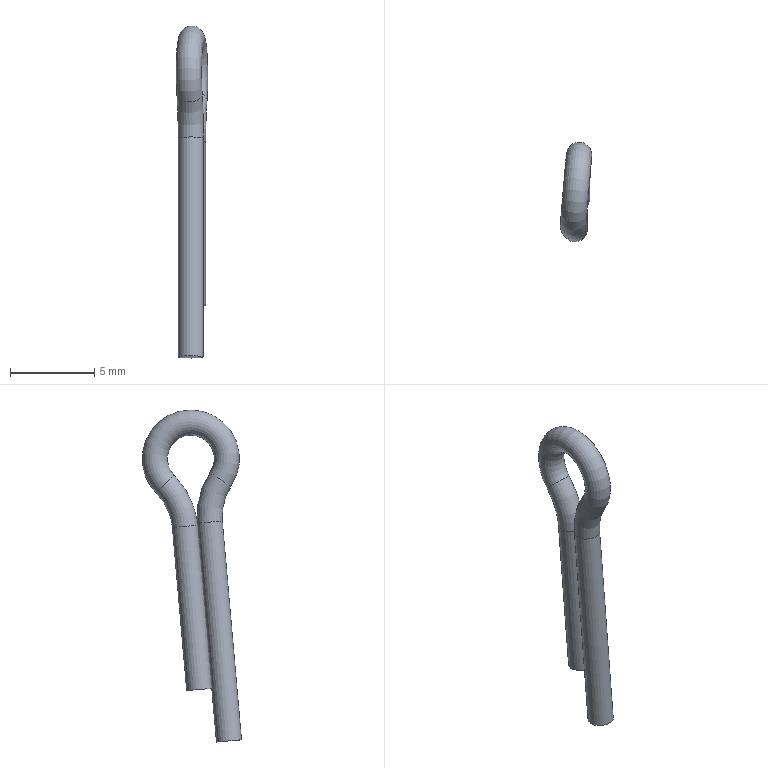Component | NX | COTTER_PIN | 1 solid | 7 faces | box 1.87 x 5.91 x 19.73 mm | volume 67 mm3 | torus 3 | cylinder 2 | plane 2 | commonest cylinder face diameters 1.5 x2
STEP:
#1=CARTESIAN_POINT('',(0.,0.,0.));
#2=DIRECTION('',(0.,0.,1.));
#3=DIRECTION('',(1.,0.,0.));
#4=AXIS2_PLACEMENT_3D('',#1,#2,#3);
#5=CARTESIAN_POINT('',(276.072,467.87,-17.811));
#6=VERTEX_POINT('',#5);
#7=CARTESIAN_POINT('',(276.006,467.126,-17.746));
#8=DIRECTION('',(0.,-0.08716,-0.9962));
#9=DIRECTION('',(0.08716,0.9924,-0.08682));
#10=AXIS2_PLACEMENT_3D('',#7,#8,#9);
#11=CIRCLE('',#10,0.75);
#12=CARTESIAN_POINT('',(276.006,467.126,-17.746));
#13=DIRECTION('',(0.,-0.08716,-0.9962));
#14=DIRECTION('',(0.08716,0.9924,-0.08682));
#15=AXIS2_PLACEMENT_3D('',#12,#13,#14);
#16=CYLINDRICAL_SURFACE('',#15,0.75);
#17=CARTESIAN_POINT('',(0.,-0.));
#18=DIRECTION('',(1.,0.));
#19=VECTOR('',#18,1.);
#20=LINE('',#17,#19);
#21=(GEOMETRIC_REPRESENTATION_CONTEXT(2)PARAMETRIC_REPRESENTATION_CONTEXT()REPRESENTATION_CONTEXT('',''));
#22=DEFINITIONAL_REPRESENTATION('',(#20),#21);
#23=PCURVE('',#16,#22);
#24=CARTESIAN_POINT('',(276.355,471.095,-18.094));
#25=DIRECTION('',(0.9962,-0.08682,0.007596));
#26=DIRECTION('',(0.,-0.08716,-0.9962));
#27=AXIS2_PLACEMENT_3D('',#24,#25,#26);
#28=TOROIDAL_SURFACE('',#27,4.,0.75);
#29=CARTESIAN_POINT('',(4.712,9.425));
#30=DIRECTION('',(0.,-1.));
#31=VECTOR('',#30,1.);
#32=LINE('',#29,#31);
#33=(GEOMETRIC_REPRESENTATION_CONTEXT(2)PARAMETRIC_REPRESENTATION_CONTEXT()REPRESENTATION_CONTEXT('',''));
#34=DEFINITIONAL_REPRESENTATION('',(#32),#33);
#35=PCURVE('',#28,#34);
#36=SURFACE_CURVE('',#11,(#23,#35),.PCURVE_S1.);
#37=EDGE_CURVE('',#6,#6,#36,.T.);
#38=ORIENTED_EDGE('',*,*,#37,.T.);
#39=CARTESIAN_POINT('',(276.072,467.022,-27.508));
#40=VERTEX_POINT('',#39);
#41=CARTESIAN_POINT('',(276.072,467.87,-17.811));
#42=CARTESIAN_POINT('',(276.072,467.022,-27.508));
#43=B_SPLINE_CURVE_WITH_KNOTS('',1,(#41,#42),.UNSPECIFIED.,.F.,.F.,(2,2),(-0.,9.734),.PIECEWISE_BEZIER_KNOTS.);
#44=CARTESIAN_POINT('',(6.283,0.));
#45=DIRECTION('',(0.,1.));
#46=VECTOR('',#45,1.);
#47=LINE('',#44,#46);
#48=(GEOMETRIC_REPRESENTATION_CONTEXT(2)PARAMETRIC_REPRESENTATION_CONTEXT()REPRESENTATION_CONTEXT('',''));
#49=DEFINITIONAL_REPRESENTATION('',(#47),#48);
#50=PCURVE('',#16,#49);
#51=CARTESIAN_POINT('',(0.,0.));
#52=DIRECTION('',(0.,1.));
#53=VECTOR('',#52,1.);
#54=LINE('',#51,#53);
#55=(GEOMETRIC_REPRESENTATION_CONTEXT(2)PARAMETRIC_REPRESENTATION_CONTEXT()REPRESENTATION_CONTEXT('',''));
#56=DEFINITIONAL_REPRESENTATION('',(#54),#55);
#57=PCURVE('',#16,#56);
#58=SEAM_CURVE('',#43,(#50,#57),.PCURVE_S1.);
#59=EDGE_CURVE('',#6,#40,#58,.T.);
#60=ORIENTED_EDGE('',*,*,#59,.T.);
#61=CARTESIAN_POINT('',(276.006,466.277,-27.443));
#62=DIRECTION('',(0.,-0.08716,-0.9962));
#63=DIRECTION('',(0.08716,0.9924,-0.08682));
#64=AXIS2_PLACEMENT_3D('',#61,#62,#63);
#65=CIRCLE('',#64,0.75);
#66=CARTESIAN_POINT('',(0.,9.734));
#67=DIRECTION('',(1.,0.));
#68=VECTOR('',#67,1.);
#69=LINE('',#66,#68);
#70=(GEOMETRIC_REPRESENTATION_CONTEXT(2)PARAMETRIC_REPRESENTATION_CONTEXT()REPRESENTATION_CONTEXT('',''));
#71=DEFINITIONAL_REPRESENTATION('',(#69),#70);
#72=PCURVE('',#16,#71);
#73=CARTESIAN_POINT('',(276.006,466.277,-27.443));
#74=DIRECTION('',(0.,-0.08716,-0.9962));
#75=DIRECTION('',(0.08716,0.9924,-0.08682));
#76=AXIS2_PLACEMENT_3D('',#73,#74,#75);
#77=PLANE('',#76);
#78=CARTESIAN_POINT('',(0.,0.));
#79=DIRECTION('',(1.,0.));
#80=AXIS2_PLACEMENT_2D('',#78,#79);
#81=CIRCLE('',#80,0.75);
#82=(GEOMETRIC_REPRESENTATION_CONTEXT(2)PARAMETRIC_REPRESENTATION_CONTEXT()REPRESENTATION_CONTEXT('',''));
#83=DEFINITIONAL_REPRESENTATION('',(#81),#82);
#84=PCURVE('',#77,#83);
#85=SURFACE_CURVE('',#65,(#72,#84),.PCURVE_S1.);
#86=EDGE_CURVE('',#40,#40,#85,.T.);
#87=ORIENTED_EDGE('',*,*,#86,.F.);
#88=ORIENTED_EDGE('',*,*,#59,.F.);
#89=EDGE_LOOP('',(#38,#60,#87,#88));
#90=FACE_BOUND('',#89,.T.);
#91=ADVANCED_FACE('',(#90),#16,.T.);
#92=CARTESIAN_POINT('',(276.139,468.813,-15.79));
#93=VERTEX_POINT('',#92);
#94=CARTESIAN_POINT('',(276.089,468.286,-15.258));
#95=DIRECTION('',(-0.05621,-0.7067,-0.7053));
#96=DIRECTION('',(0.06661,0.7022,-0.7088));
#97=AXIS2_PLACEMENT_3D('',#94,#95,#96);
#98=CIRCLE('',#97,0.75);
#99=CARTESIAN_POINT('',(4.011,9.425));
#100=DIRECTION('',(0.,-1.));
#101=VECTOR('',#100,1.);
#102=LINE('',#99,#101);
#103=(GEOMETRIC_REPRESENTATION_CONTEXT(2)PARAMETRIC_REPRESENTATION_CONTEXT()REPRESENTATION_CONTEXT('',''));
#104=DEFINITIONAL_REPRESENTATION('',(#102),#103);
#105=PCURVE('',#28,#104);
#106=CARTESIAN_POINT('',(275.945,466.777,-13.734));
#107=DIRECTION('',(-0.9962,0.08682,-0.007596));
#108=DIRECTION('',(-0.,0.08716,0.9962));
#109=AXIS2_PLACEMENT_3D('',#106,#107,#108);
#110=TOROIDAL_SURFACE('',#109,2.15,0.75);
#111=CARTESIAN_POINT('',(8.555,6.283));
#112=DIRECTION('',(0.,-1.));
#113=VECTOR('',#112,1.);
#114=LINE('',#111,#113);
#115=(GEOMETRIC_REPRESENTATION_CONTEXT(2)PARAMETRIC_REPRESENTATION_CONTEXT()REPRESENTATION_CONTEXT('',''));
#116=DEFINITIONAL_REPRESENTATION('',(#114),#115);
#117=PCURVE('',#110,#116);
#118=SURFACE_CURVE('',#98,(#105,#117),.PCURVE_S1.);
#119=EDGE_CURVE('',#93,#93,#118,.T.);
#120=ORIENTED_EDGE('',*,*,#119,.T.);
#121=CARTESIAN_POINT('',(276.139,468.813,-15.79));
#122=CARTESIAN_POINT('',(276.117,468.544,-16.059));
#123=CARTESIAN_POINT('',(276.099,468.313,-16.364));
#124=CARTESIAN_POINT('',(276.086,468.127,-16.7));
#125=CARTESIAN_POINT('',(276.077,467.989,-17.058));
#126=CARTESIAN_POINT('',(276.072,467.903,-17.432));
#127=CARTESIAN_POINT('',(276.072,467.87,-17.811));
#128=(BOUNDED_CURVE()B_SPLINE_CURVE(6,(#121,#122,#123,#124,#125,#126,#127),.UNSPECIFIED.,.F.,.F.)B_SPLINE_CURVE_WITH_KNOTS((7,7),(4.011,4.712),.PIECEWISE_BEZIER_KNOTS.)CURVE()GEOMETRIC_REPRESENTATION_ITEM()RATIONAL_B_SPLINE_CURVE((1.006,1.002,0.9996,0.9988,0.9996,1.002,1.006))REPRESENTATION_ITEM(''));
#129=CARTESIAN_POINT('',(0.,3.142));
#130=DIRECTION('',(1.,0.));
#131=VECTOR('',#130,1.);
#132=LINE('',#129,#131);
#133=(GEOMETRIC_REPRESENTATION_CONTEXT(2)PARAMETRIC_REPRESENTATION_CONTEXT()REPRESENTATION_CONTEXT('',''));
#134=DEFINITIONAL_REPRESENTATION('',(#132),#133);
#135=PCURVE('',#28,#134);
#136=CARTESIAN_POINT('',(0.,9.425));
#137=DIRECTION('',(1.,0.));
#138=VECTOR('',#137,1.);
#139=LINE('',#136,#138);
#140=(GEOMETRIC_REPRESENTATION_CONTEXT(2)PARAMETRIC_REPRESENTATION_CONTEXT()REPRESENTATION_CONTEXT('',''));
#141=DEFINITIONAL_REPRESENTATION('',(#139),#140);
#142=PCURVE('',#28,#141);
#143=SEAM_CURVE('',#128,(#135,#142),.PCURVE_S1.);
#144=EDGE_CURVE('',#93,#6,#143,.T.);
#145=ORIENTED_EDGE('',*,*,#144,.T.);
#146=ORIENTED_EDGE('',*,*,#37,.F.);
#147=ORIENTED_EDGE('',*,*,#144,.F.);
#148=EDGE_LOOP('',(#120,#145,#146,#147));
#149=FACE_BOUND('',#148,.T.);
#150=ADVANCED_FACE('',(#149),#28,.T.);
#151=CARTESIAN_POINT('',(275.748,464.372,-15.344));
#152=VERTEX_POINT('',#151);
#153=CARTESIAN_POINT('',(275.799,464.994,-14.927));
#154=DIRECTION('',(-0.05449,-0.5524,0.8318));
#155=DIRECTION('',(-0.06802,-0.829,-0.555));
#156=AXIS2_PLACEMENT_3D('',#153,#154,#155);
#157=CIRCLE('',#156,0.75);
#158=CARTESIAN_POINT('',(4.037,6.283));
#159=DIRECTION('',(0.,-1.));
#160=VECTOR('',#159,1.);
#161=LINE('',#158,#160);
#162=(GEOMETRIC_REPRESENTATION_CONTEXT(2)PARAMETRIC_REPRESENTATION_CONTEXT()REPRESENTATION_CONTEXT('',''));
#163=DEFINITIONAL_REPRESENTATION('',(#161),#162);
#164=PCURVE('',#110,#163);
#165=CARTESIAN_POINT('',(275.527,461.678,-17.148));
#166=DIRECTION('',(0.9962,-0.08682,0.007596));
#167=DIRECTION('',(0.,-0.08716,-0.9962));
#168=AXIS2_PLACEMENT_3D('',#165,#166,#167);
#169=TOROIDAL_SURFACE('',#168,4.,0.75);
#170=CARTESIAN_POINT('',(8.529,9.425));
#171=DIRECTION('',(0.,-1.));
#172=VECTOR('',#171,1.);
#173=LINE('',#170,#172);
#174=(GEOMETRIC_REPRESENTATION_CONTEXT(2)PARAMETRIC_REPRESENTATION_CONTEXT()REPRESENTATION_CONTEXT('',''));
#175=DEFINITIONAL_REPRESENTATION('',(#173),#174);
#176=PCURVE('',#169,#175);
#177=SURFACE_CURVE('',#157,(#164,#176),.PCURVE_S1.);
#178=EDGE_CURVE('',#152,#152,#177,.T.);
#179=ORIENTED_EDGE('',*,*,#178,.T.);
#180=CARTESIAN_POINT('',(275.748,464.372,-15.344));
#181=CARTESIAN_POINT('',(275.677,463.649,-14.254));
#182=CARTESIAN_POINT('',(275.65,463.47,-12.799));
#183=CARTESIAN_POINT('',(275.689,464.042,-11.288));
#184=CARTESIAN_POINT('',(275.796,465.37,-10.163));
#185=CARTESIAN_POINT('',(275.95,467.167,-9.848));
#186=CARTESIAN_POINT('',(276.103,468.865,-10.514));
#187=CARTESIAN_POINT('',(276.207,469.942,-11.881));
#188=CARTESIAN_POINT('',(276.242,470.203,-13.475));
#189=CARTESIAN_POINT('',(276.212,469.739,-14.866));
#190=CARTESIAN_POINT('',(276.139,468.813,-15.79));
#191=B_SPLINE_CURVE_WITH_KNOTS('',10,(#180,#181,#182,#183,#184,#185,#186,#187,#188,#189,#190),.UNSPECIFIED.,.F.,.F.,(11,11),(4.037,8.555),.PIECEWISE_BEZIER_KNOTS.);
#192=CARTESIAN_POINT('',(0.,0.));
#193=DIRECTION('',(1.,0.));
#194=VECTOR('',#193,1.);
#195=LINE('',#192,#194);
#196=(GEOMETRIC_REPRESENTATION_CONTEXT(2)PARAMETRIC_REPRESENTATION_CONTEXT()REPRESENTATION_CONTEXT('',''));
#197=DEFINITIONAL_REPRESENTATION('',(#195),#196);
#198=PCURVE('',#110,#197);
#199=CARTESIAN_POINT('',(0.,6.283));
#200=DIRECTION('',(1.,0.));
#201=VECTOR('',#200,1.);
#202=LINE('',#199,#201);
#203=(GEOMETRIC_REPRESENTATION_CONTEXT(2)PARAMETRIC_REPRESENTATION_CONTEXT()REPRESENTATION_CONTEXT('',''));
#204=DEFINITIONAL_REPRESENTATION('',(#202),#203);
#205=PCURVE('',#110,#204);
#206=SEAM_CURVE('',#191,(#198,#205),.PCURVE_S1.);
#207=EDGE_CURVE('',#152,#93,#206,.T.);
#208=ORIENTED_EDGE('',*,*,#207,.T.);
#209=ORIENTED_EDGE('',*,*,#119,.F.);
#210=ORIENTED_EDGE('',*,*,#207,.F.);
#211=EDGE_LOOP('',(#179,#208,#209,#210));
#212=FACE_BOUND('',#211,.T.);
#213=ADVANCED_FACE('',(#212),#110,.T.);
#214=CARTESIAN_POINT('',(275.81,464.903,-17.43));
#215=VERTEX_POINT('',#214);
#216=CARTESIAN_POINT('',(275.876,465.648,-17.495));
#217=DIRECTION('',(-0.,0.08716,0.9962));
#218=DIRECTION('',(-0.08716,-0.9924,0.08682));
#219=AXIS2_PLACEMENT_3D('',#216,#217,#218);
#220=CIRCLE('',#219,0.75);
#221=CARTESIAN_POINT('',(7.854,9.425));
#222=DIRECTION('',(0.,-1.));
#223=VECTOR('',#222,1.);
#224=LINE('',#221,#223);
#225=(GEOMETRIC_REPRESENTATION_CONTEXT(2)PARAMETRIC_REPRESENTATION_CONTEXT()REPRESENTATION_CONTEXT('',''));
#226=DEFINITIONAL_REPRESENTATION('',(#224),#225);
#227=PCURVE('',#169,#226);
#228=CARTESIAN_POINT('',(275.876,464.789,-27.313));
#229=DIRECTION('',(0.,-0.08716,-0.9962));
#230=DIRECTION('',(0.08716,0.9924,-0.08682));
#231=AXIS2_PLACEMENT_3D('',#228,#229,#230);
#232=CYLINDRICAL_SURFACE('',#231,0.75);
#233=CARTESIAN_POINT('',(9.425,-9.855));
#234=DIRECTION('',(-1.,0.));
#235=VECTOR('',#234,1.);
#236=LINE('',#233,#235);
#237=(GEOMETRIC_REPRESENTATION_CONTEXT(2)PARAMETRIC_REPRESENTATION_CONTEXT()REPRESENTATION_CONTEXT('',''));
#238=DEFINITIONAL_REPRESENTATION('',(#236),#237);
#239=PCURVE('',#232,#238);
#240=SURFACE_CURVE('',#220,(#227,#239),.PCURVE_S1.);
#241=EDGE_CURVE('',#215,#215,#240,.T.);
#242=ORIENTED_EDGE('',*,*,#241,.T.);
#243=CARTESIAN_POINT('',(275.81,464.903,-17.43));
#244=CARTESIAN_POINT('',(275.81,464.935,-17.064));
#245=CARTESIAN_POINT('',(275.806,464.918,-16.695));
#246=CARTESIAN_POINT('',(275.797,464.851,-16.332));
#247=CARTESIAN_POINT('',(275.785,464.736,-15.981));
#248=CARTESIAN_POINT('',(275.768,464.575,-15.649));
#249=CARTESIAN_POINT('',(275.748,464.372,-15.344));
#250=(BOUNDED_CURVE()B_SPLINE_CURVE(6,(#243,#244,#245,#246,#247,#248,#249),.UNSPECIFIED.,.F.,.F.)B_SPLINE_CURVE_WITH_KNOTS((7,7),(1.571,2.246),.PIECEWISE_BEZIER_KNOTS.)CURVE()GEOMETRIC_REPRESENTATION_ITEM()RATIONAL_B_SPLINE_CURVE((1.006,1.002,0.9996,0.9989,0.9996,1.002,1.006))REPRESENTATION_ITEM(''));
#251=CARTESIAN_POINT('',(6.283,3.142));
#252=DIRECTION('',(1.,0.));
#253=VECTOR('',#252,1.);
#254=LINE('',#251,#253);
#255=(GEOMETRIC_REPRESENTATION_CONTEXT(2)PARAMETRIC_REPRESENTATION_CONTEXT()REPRESENTATION_CONTEXT('',''));
#256=DEFINITIONAL_REPRESENTATION('',(#254),#255);
#257=PCURVE('',#169,#256);
#258=CARTESIAN_POINT('',(6.283,9.425));
#259=DIRECTION('',(1.,0.));
#260=VECTOR('',#259,1.);
#261=LINE('',#258,#260);
#262=(GEOMETRIC_REPRESENTATION_CONTEXT(2)PARAMETRIC_REPRESENTATION_CONTEXT()REPRESENTATION_CONTEXT('',''));
#263=DEFINITIONAL_REPRESENTATION('',(#261),#262);
#264=PCURVE('',#169,#263);
#265=SEAM_CURVE('',#250,(#257,#264),.PCURVE_S1.);
#266=EDGE_CURVE('',#215,#152,#265,.T.);
#267=ORIENTED_EDGE('',*,*,#266,.T.);
#268=ORIENTED_EDGE('',*,*,#178,.F.);
#269=ORIENTED_EDGE('',*,*,#266,.F.);
#270=EDGE_LOOP('',(#242,#267,#268,#269));
#271=FACE_BOUND('',#270,.T.);
#272=ADVANCED_FACE('',(#271),#169,.T.);
#273=CARTESIAN_POINT('',(275.81,463.765,-30.435));
#274=VERTEX_POINT('',#273);
#275=CARTESIAN_POINT('',(275.876,464.51,-30.5));
#276=DIRECTION('',(-0.,0.08716,0.9962));
#277=DIRECTION('',(-0.08716,-0.9924,0.08682));
#278=AXIS2_PLACEMENT_3D('',#275,#276,#277);
#279=CIRCLE('',#278,0.75);
#280=CARTESIAN_POINT('',(9.425,3.2));
#281=DIRECTION('',(-1.,0.));
#282=VECTOR('',#281,1.);
#283=LINE('',#280,#282);
#284=(GEOMETRIC_REPRESENTATION_CONTEXT(2)PARAMETRIC_REPRESENTATION_CONTEXT()REPRESENTATION_CONTEXT('',''));
#285=DEFINITIONAL_REPRESENTATION('',(#283),#284);
#286=PCURVE('',#232,#285);
#287=CARTESIAN_POINT('',(275.876,464.51,-30.5));
#288=DIRECTION('',(-0.,0.08716,0.9962));
#289=DIRECTION('',(-0.08716,-0.9924,0.08682));
#290=AXIS2_PLACEMENT_3D('',#287,#288,#289);
#291=PLANE('',#290);
#292=CARTESIAN_POINT('',(0.,0.));
#293=DIRECTION('',(1.,-0.));
#294=AXIS2_PLACEMENT_2D('',#292,#293);
#295=CIRCLE('',#294,0.75);
#296=(GEOMETRIC_REPRESENTATION_CONTEXT(2)PARAMETRIC_REPRESENTATION_CONTEXT()REPRESENTATION_CONTEXT('',''));
#297=DEFINITIONAL_REPRESENTATION('',(#295),#296);
#298=PCURVE('',#291,#297);
#299=SURFACE_CURVE('',#279,(#286,#298),.PCURVE_S1.);
#300=EDGE_CURVE('',#274,#274,#299,.T.);
#301=ORIENTED_EDGE('',*,*,#300,.T.);
#302=CARTESIAN_POINT('',(275.81,464.903,-17.43));
#303=CARTESIAN_POINT('',(275.81,463.765,-30.435));
#304=B_SPLINE_CURVE_WITH_KNOTS('',1,(#302,#303),.UNSPECIFIED.,.F.,.F.,(2,2),(-9.855,3.2),.PIECEWISE_BEZIER_KNOTS.);
#305=CARTESIAN_POINT('',(3.142,0.));
#306=DIRECTION('',(0.,1.));
#307=VECTOR('',#306,1.);
#308=LINE('',#305,#307);
#309=(GEOMETRIC_REPRESENTATION_CONTEXT(2)PARAMETRIC_REPRESENTATION_CONTEXT()REPRESENTATION_CONTEXT('',''));
#310=DEFINITIONAL_REPRESENTATION('',(#308),#309);
#311=PCURVE('',#232,#310);
#312=CARTESIAN_POINT('',(9.425,0.));
#313=DIRECTION('',(0.,1.));
#314=VECTOR('',#313,1.);
#315=LINE('',#312,#314);
#316=(GEOMETRIC_REPRESENTATION_CONTEXT(2)PARAMETRIC_REPRESENTATION_CONTEXT()REPRESENTATION_CONTEXT('',''));
#317=DEFINITIONAL_REPRESENTATION('',(#315),#316);
#318=PCURVE('',#232,#317);
#319=SEAM_CURVE('',#304,(#311,#318),.PCURVE_S1.);
#320=EDGE_CURVE('',#215,#274,#319,.T.);
#321=ORIENTED_EDGE('',*,*,#320,.F.);
#322=ORIENTED_EDGE('',*,*,#241,.F.);
#323=ORIENTED_EDGE('',*,*,#320,.T.);
#324=EDGE_LOOP('',(#301,#321,#322,#323));
#325=FACE_BOUND('',#324,.T.);
#326=ADVANCED_FACE('',(#325),#232,.T.);
#327=ORIENTED_EDGE('',*,*,#86,.T.);
#328=EDGE_LOOP('',(#327));
#329=FACE_BOUND('',#328,.T.);
#330=ADVANCED_FACE('',(#329),#77,.T.);
#331=ORIENTED_EDGE('',*,*,#300,.F.);
#332=EDGE_LOOP('',(#331));
#333=FACE_BOUND('',#332,.T.);
#334=ADVANCED_FACE('',(#333),#291,.F.);
#335=CLOSED_SHELL('',(#91,#150,#213,#272,#326,#330,#334));
#336=MANIFOLD_SOLID_BREP('',#335);
#337=(LENGTH_UNIT()NAMED_UNIT(*)SI_UNIT(.MILLI.,.METRE.));
#338=UNCERTAINTY_MEASURE_WITH_UNIT(LENGTH_MEASURE(0.00001),#337,'','');
#339=(NAMED_UNIT(*)PLANE_ANGLE_UNIT()SI_UNIT($,.RADIAN.));
#340=(NAMED_UNIT(*)SI_UNIT($,.STERADIAN.)SOLID_ANGLE_UNIT());
#341=(GEOMETRIC_REPRESENTATION_CONTEXT(3)GLOBAL_UNCERTAINTY_ASSIGNED_CONTEXT((#338))GLOBAL_UNIT_ASSIGNED_CONTEXT((#337,#339,#340))REPRESENTATION_CONTEXT('',''));
#342=ADVANCED_BREP_SHAPE_REPRESENTATION('',(#4,#336),#341);